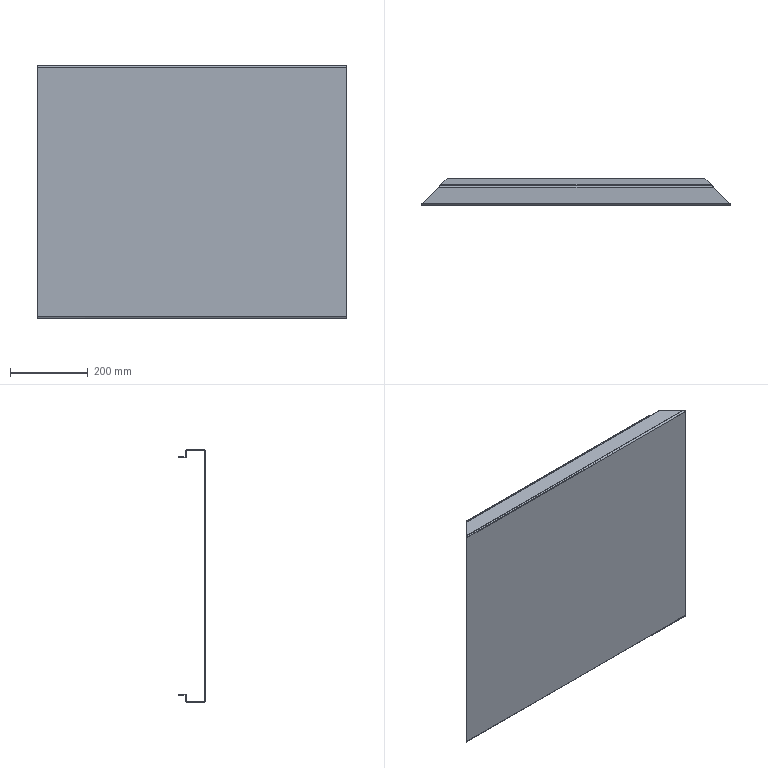Component | SolidWorks | BoxWelding-1_UpperAndLowerPlate-1 | 1 solid | 54 faces | volume 1266578 mm3 | plane 30 | cylinder 12 | spline 12 | commonest cylinder face diameters 8 x6 4 x6